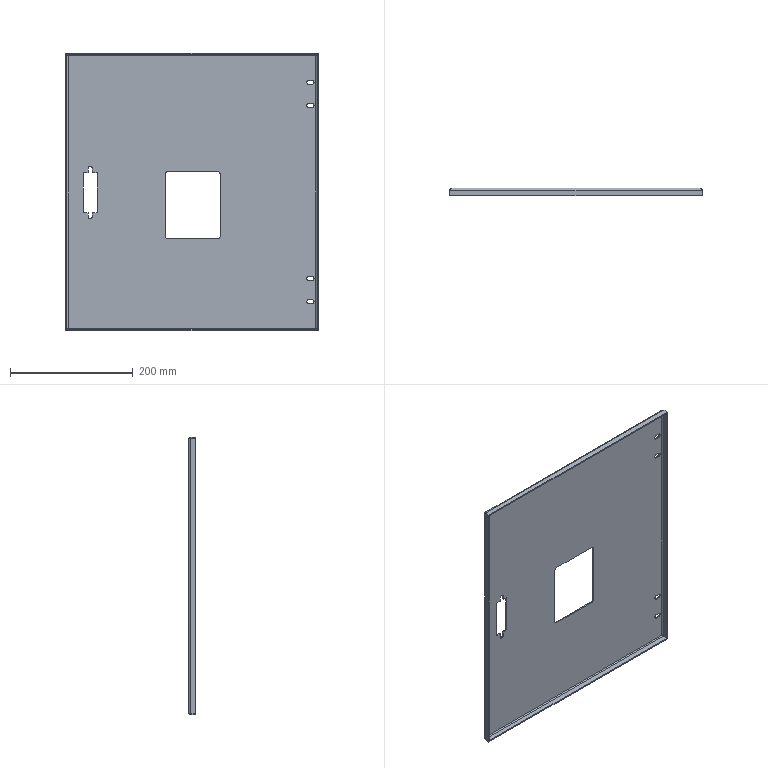Component | SolidWorks | ElectricalCabinetAssembly-1_BreakerDoor-2 | 1 solid | 78 faces | volume 379626 mm3 | plane 44 | cylinder 26 | spline 8 | commonest cylinder face diameters 7 x14 4 x4 8 x4 10 x4 | material Plain Carbon Steel